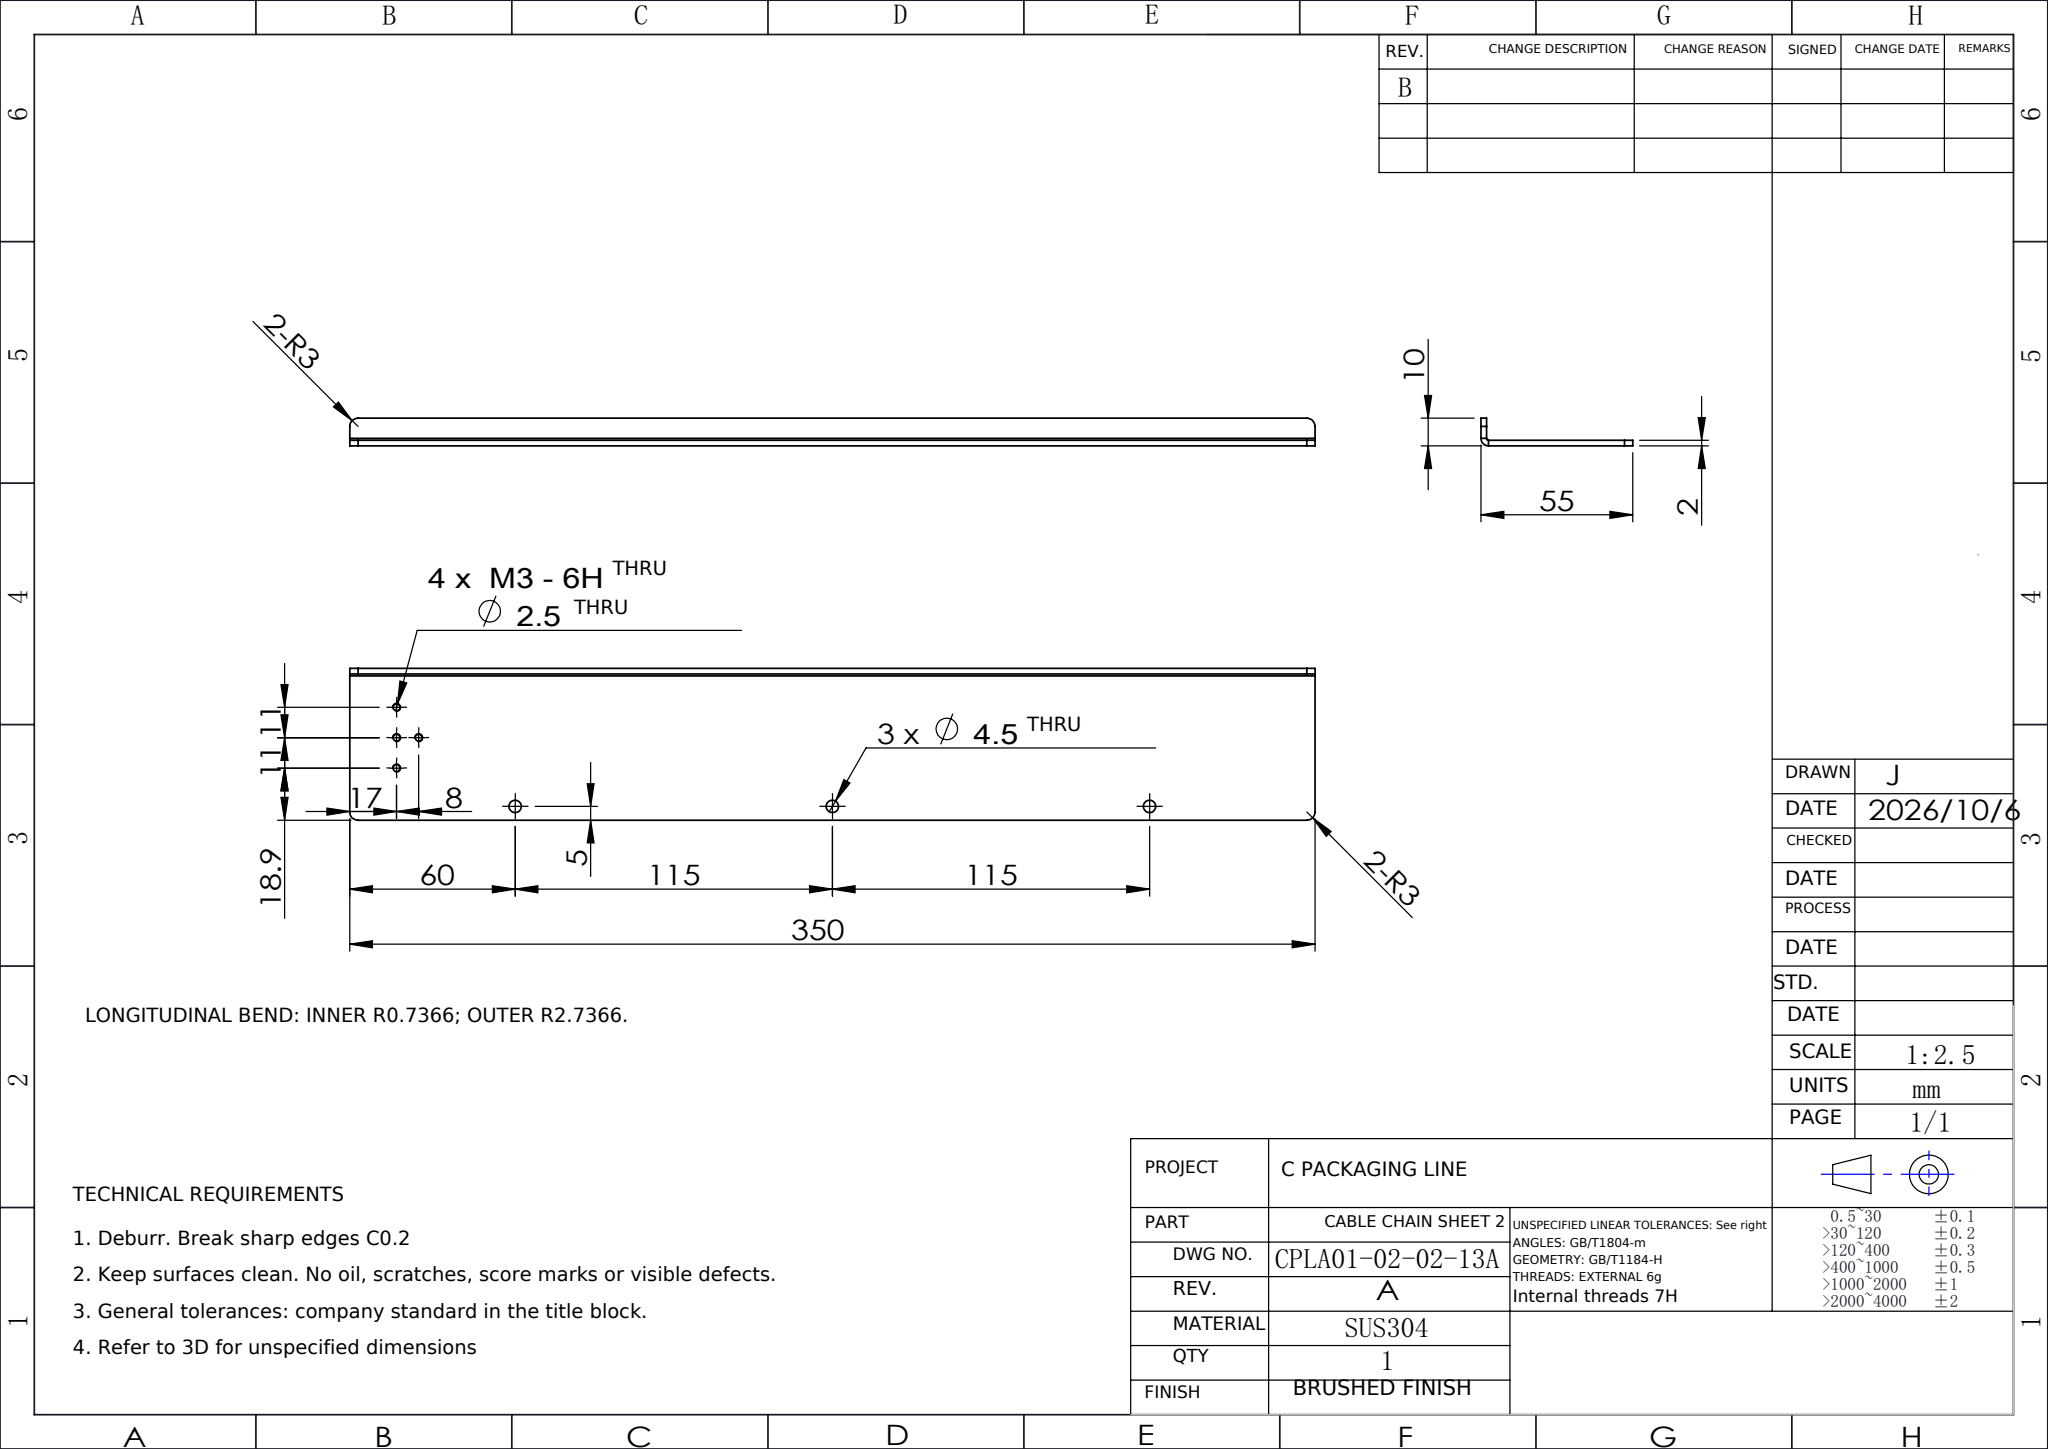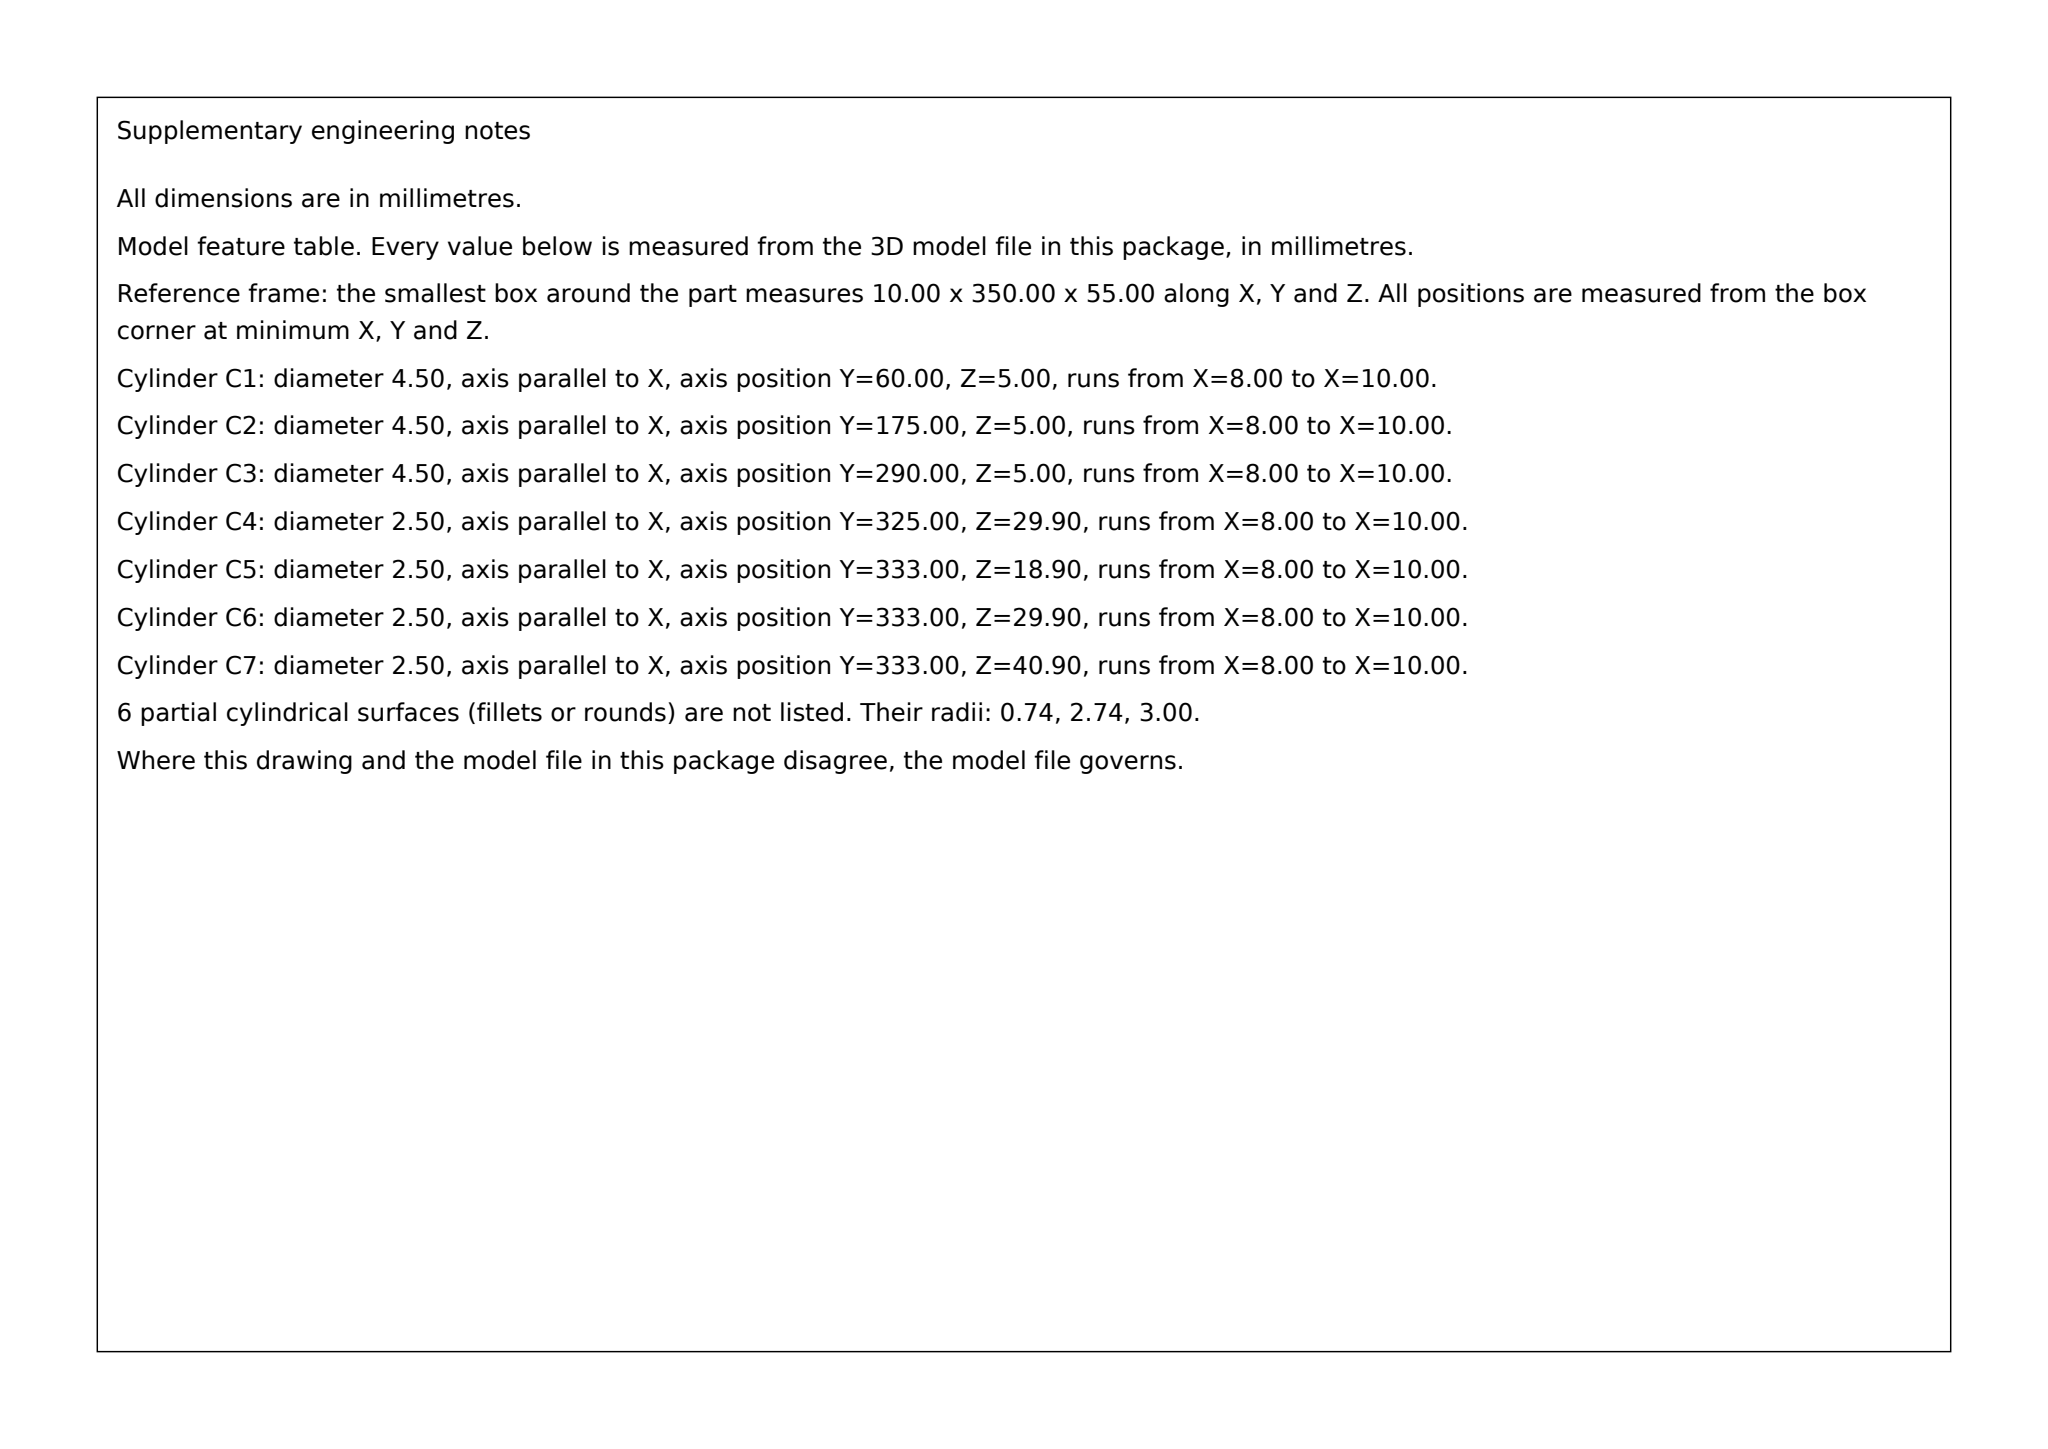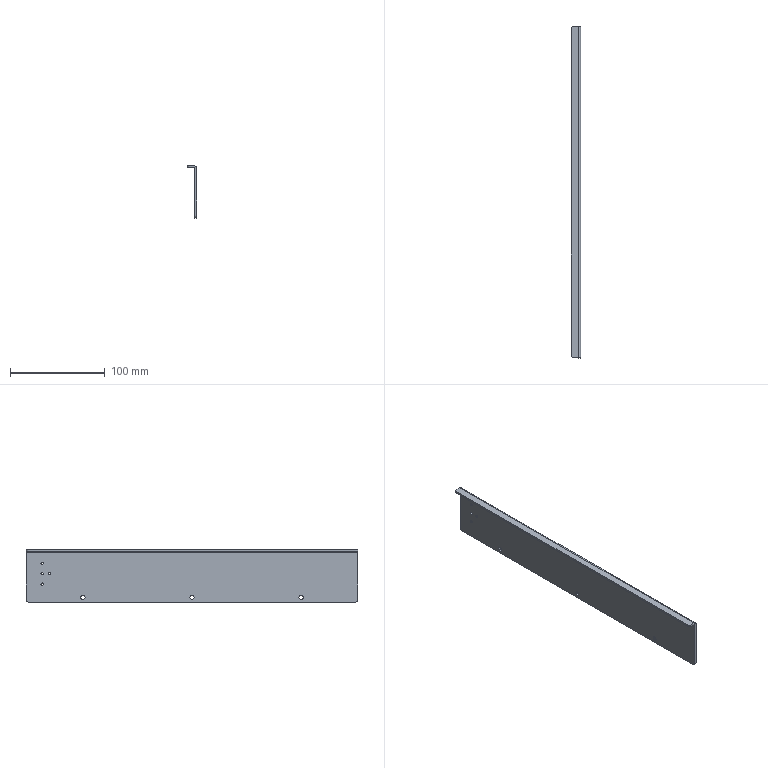Part | SolidWorks | mm | 1 solid | 32 faces | box 10 x 350 x 55 mm | volume 43428 mm3 | cylinder 20 | plane 12 | commonest cylinder face diameters 2.5 x8 4.5 x6 6 x4 5.473 x1 1.473 x1